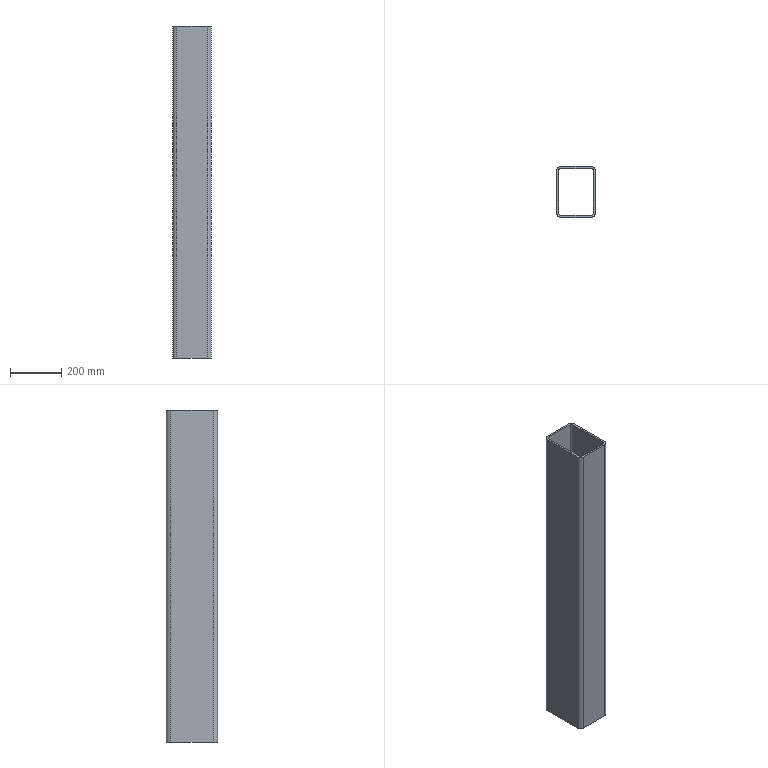Component | NX | AAAAAAAAAAAAAAAAAAAAAAAAAAAAAAAAAAAAAAAAAAAAAAAAAAAAAAAAAAA_10 | 1 solid | 18 faces | volume 6732942 mm3 | plane 10 | cylinder 8 | commonest cylinder face diameters 32 x4 16 x4